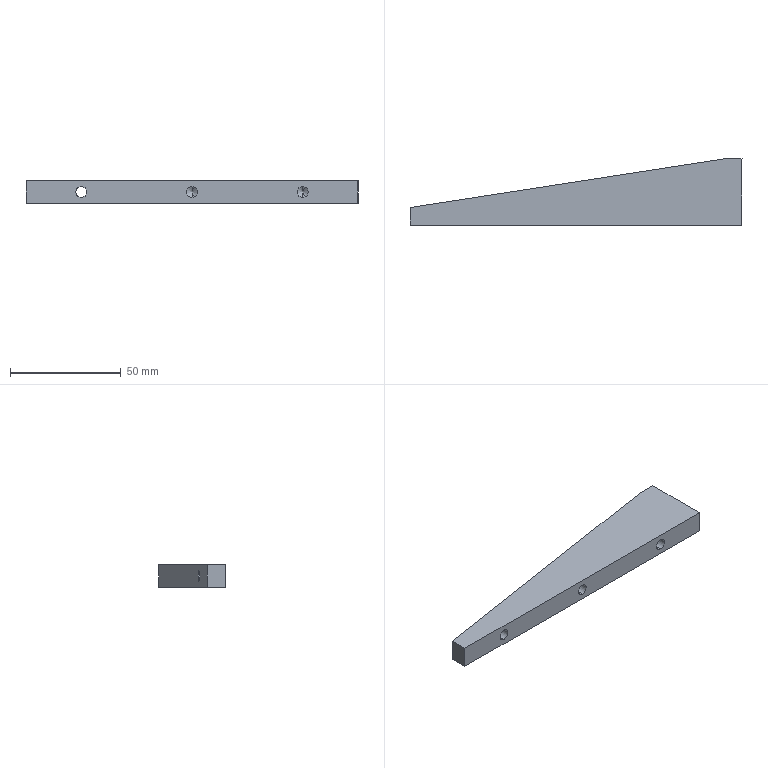Component | SolidWorks | 17081801-804-026A-1 | 1 solid | 25 faces | box 150 x 30 x 10 mm | volume 27929 mm3 | cylinder 10 | cone 8 | plane 7 | commonest cylinder face diameters 5 x10 | material AL6061
build123d program:
from build123d import *

# Parameters (mm, degrees)
BOSS_EXTRUDE1_DEPTH   = 5
M6_TAPPED_HOLE1_D     = 5
M6_TAPPED_HOLE1_DEPTH = 15
M6_TAPPED_HOLE1_TIP   = 1.502
M6_TAPPED_HOLE2_D     = 5
M6_TAPPED_HOLE2_DEPTH = 15
M6_TAPPED_HOLE2_TIP   = 1.502


with BuildPart() as part:
    # Sketch1 → Boss-Extrude1 (new, symmetric)
    with BuildSketch(Plane.XY):
        Polygon((0, 0), (0, 150), (-8, 150), (-30, 8), (-30, 0), align=None)
    extrude(amount=BOSS_EXTRUDE1_DEPTH, both=True)

    # M6 Tapped Hole1
    with Locations(Plane(origin=(0, 0, 0), x_dir=(0, 0, -1), z_dir=(1, 0, 0))):
        with Locations((0, 25), (0, 75), (0, 125)):
            Hole(M6_TAPPED_HOLE1_D / 2, depth=M6_TAPPED_HOLE1_DEPTH)
            with Locations((0, 0, -(M6_TAPPED_HOLE1_DEPTH + M6_TAPPED_HOLE1_TIP / 2))):  # 118° drill point
                Cone(0, M6_TAPPED_HOLE1_D / 2, M6_TAPPED_HOLE1_TIP, mode=Mode.SUBTRACT)

    # M6 Tapped Hole2
    with Locations(Plane(origin=(0, 0, 0), x_dir=(-1, 0, 0), z_dir=(0, -1, 0))):
        with Locations((25, 0), (10, 0)):
            Hole(M6_TAPPED_HOLE2_D / 2, depth=M6_TAPPED_HOLE2_DEPTH)
            with Locations((0, 0, -(M6_TAPPED_HOLE2_DEPTH + M6_TAPPED_HOLE2_TIP / 2))):  # 118° drill point
                Cone(0, M6_TAPPED_HOLE2_D / 2, M6_TAPPED_HOLE2_TIP, mode=Mode.SUBTRACT)


solid = part.part

# Placed as in the assembly
solid = solid.moved(Location((237, 2110.4, 171), (180, 0, 90)))
STEP:
#1=CARTESIAN_POINT('',(8.74,84.071,6.634));
#2=VERTEX_POINT('',#1);
#3=CARTESIAN_POINT('',(8.74,84.071,6.831));
#4=VERTEX_POINT('',#3);
#5=CARTESIAN_POINT('',(8.74,84.071,6.732));
#6=DIRECTION('',(1.,-0.,0.));
#7=DIRECTION('',(0.,0.,1.));
#8=AXIS2_PLACEMENT_3D('',#5,#6,#7);
#9=CIRCLE('',#8,0.09843);
#10=EDGE_CURVE('',#2,#4,#9,.T.);
#11=ORIENTED_EDGE('',*,*,#10,.F.);
#12=CARTESIAN_POINT('',(9.331,84.071,6.634));
#13=VERTEX_POINT('',#12);
#14=CARTESIAN_POINT('',(9.331,84.071,6.634));
#15=DIRECTION('',(1.,-0.,0.));
#16=VECTOR('',#15,39.37);
#17=LINE('',#14,#16);
#18=EDGE_CURVE('',#2,#13,#17,.T.);
#19=ORIENTED_EDGE('',*,*,#18,.T.);
#20=CARTESIAN_POINT('',(9.331,84.071,6.831));
#21=VERTEX_POINT('',#20);
#22=CARTESIAN_POINT('',(9.331,84.071,6.732));
#23=DIRECTION('',(1.,-0.,0.));
#24=DIRECTION('',(0.,0.,1.));
#25=AXIS2_PLACEMENT_3D('',#22,#23,#24);
#26=CIRCLE('',#25,0.09843);
#27=EDGE_CURVE('',#13,#21,#26,.T.);
#28=ORIENTED_EDGE('',*,*,#27,.T.);
#29=CARTESIAN_POINT('',(9.331,84.071,6.831));
#30=DIRECTION('',(1.,-0.,0.));
#31=VECTOR('',#30,39.37);
#32=LINE('',#29,#31);
#33=EDGE_CURVE('',#4,#21,#32,.T.);
#34=ORIENTED_EDGE('',*,*,#33,.F.);
#35=EDGE_LOOP('',(#11,#19,#28,#34));
#36=FACE_OUTER_BOUND('',#35,.T.);
#37=CARTESIAN_POINT('',(9.331,84.071,6.732));
#38=DIRECTION('',(1.,-0.,0.));
#39=DIRECTION('',(0.,0.,1.));
#40=AXIS2_PLACEMENT_3D('',#37,#38,#39);
#41=CYLINDRICAL_SURFACE('',#40,0.09843);
#42=ADVANCED_FACE('',(#36),#41,.F.);
#43=CARTESIAN_POINT('',(8.681,84.071,6.732));
#44=VERTEX_POINT('',#43);
#45=CARTESIAN_POINT('',(8.74,84.071,6.831));
#46=DIRECTION('',(0.515,-0.,0.8572));
#47=VECTOR('',#46,39.37);
#48=LINE('',#45,#47);
#49=EDGE_CURVE('',#44,#4,#48,.T.);
#50=ORIENTED_EDGE('',*,*,#49,.F.);
#51=CARTESIAN_POINT('',(8.74,84.071,6.634));
#52=DIRECTION('',(0.515,-0.,-0.8572));
#53=VECTOR('',#52,39.37);
#54=LINE('',#51,#53);
#55=EDGE_CURVE('',#44,#2,#54,.T.);
#56=ORIENTED_EDGE('',*,*,#55,.T.);
#57=ORIENTED_EDGE('',*,*,#10,.T.);
#58=EDGE_LOOP('',(#50,#56,#57));
#59=FACE_OUTER_BOUND('',#58,.T.);
#60=CARTESIAN_POINT('',(8.74,84.071,6.732));
#61=DIRECTION('',(1.,-0.,0.));
#62=DIRECTION('',(0.,0.,1.));
#63=AXIS2_PLACEMENT_3D('',#60,#61,#62);
#64=CONICAL_SURFACE('',#63,0.09843,1.03);
#65=ADVANCED_FACE('',(#59),#64,.F.);
#66=CARTESIAN_POINT('',(8.74,83.48,6.634));
#67=VERTEX_POINT('',#66);
#68=CARTESIAN_POINT('',(8.74,83.48,6.831));
#69=VERTEX_POINT('',#68);
#70=CARTESIAN_POINT('',(8.74,83.48,6.732));
#71=DIRECTION('',(1.,-0.,0.));
#72=DIRECTION('',(0.,0.,1.));
#73=AXIS2_PLACEMENT_3D('',#70,#71,#72);
#74=CIRCLE('',#73,0.09843);
#75=EDGE_CURVE('',#67,#69,#74,.T.);
#76=ORIENTED_EDGE('',*,*,#75,.F.);
#77=CARTESIAN_POINT('',(9.331,83.48,6.634));
#78=VERTEX_POINT('',#77);
#79=CARTESIAN_POINT('',(9.331,83.48,6.634));
#80=DIRECTION('',(1.,-0.,0.));
#81=VECTOR('',#80,39.37);
#82=LINE('',#79,#81);
#83=EDGE_CURVE('',#67,#78,#82,.T.);
#84=ORIENTED_EDGE('',*,*,#83,.T.);
#85=CARTESIAN_POINT('',(9.331,83.48,6.831));
#86=VERTEX_POINT('',#85);
#87=CARTESIAN_POINT('',(9.331,83.48,6.732));
#88=DIRECTION('',(1.,-0.,0.));
#89=DIRECTION('',(0.,0.,1.));
#90=AXIS2_PLACEMENT_3D('',#87,#88,#89);
#91=CIRCLE('',#90,0.09843);
#92=EDGE_CURVE('',#78,#86,#91,.T.);
#93=ORIENTED_EDGE('',*,*,#92,.T.);
#94=CARTESIAN_POINT('',(9.331,83.48,6.831));
#95=DIRECTION('',(1.,-0.,0.));
#96=VECTOR('',#95,39.37);
#97=LINE('',#94,#96);
#98=EDGE_CURVE('',#69,#86,#97,.T.);
#99=ORIENTED_EDGE('',*,*,#98,.F.);
#100=EDGE_LOOP('',(#76,#84,#93,#99));
#101=FACE_OUTER_BOUND('',#100,.T.);
#102=CARTESIAN_POINT('',(9.331,83.48,6.732));
#103=DIRECTION('',(1.,-0.,0.));
#104=DIRECTION('',(0.,0.,1.));
#105=AXIS2_PLACEMENT_3D('',#102,#103,#104);
#106=CYLINDRICAL_SURFACE('',#105,0.09843);
#107=ADVANCED_FACE('',(#101),#106,.F.);
#108=CARTESIAN_POINT('',(8.681,83.48,6.732));
#109=VERTEX_POINT('',#108);
#110=CARTESIAN_POINT('',(8.74,83.48,6.831));
#111=DIRECTION('',(0.515,-0.,0.8572));
#112=VECTOR('',#111,39.37);
#113=LINE('',#110,#112);
#114=EDGE_CURVE('',#109,#69,#113,.T.);
#115=ORIENTED_EDGE('',*,*,#114,.F.);
#116=CARTESIAN_POINT('',(8.74,83.48,6.634));
#117=DIRECTION('',(0.515,-0.,-0.8572));
#118=VECTOR('',#117,39.37);
#119=LINE('',#116,#118);
#120=EDGE_CURVE('',#109,#67,#119,.T.);
#121=ORIENTED_EDGE('',*,*,#120,.T.);
#122=ORIENTED_EDGE('',*,*,#75,.T.);
#123=EDGE_LOOP('',(#115,#121,#122));
#124=FACE_OUTER_BOUND('',#123,.T.);
#125=CARTESIAN_POINT('',(8.74,83.48,6.732));
#126=DIRECTION('',(1.,-0.,0.));
#127=DIRECTION('',(0.,0.,1.));
#128=AXIS2_PLACEMENT_3D('',#125,#126,#127);
#129=CONICAL_SURFACE('',#128,0.09843,1.03);
#130=ADVANCED_FACE('',(#124),#129,.F.);
#131=CARTESIAN_POINT('',(8.346,83.677,6.634));
#132=VERTEX_POINT('',#131);
#133=CARTESIAN_POINT('',(8.346,83.677,6.831));
#134=VERTEX_POINT('',#133);
#135=CARTESIAN_POINT('',(8.346,83.677,6.732));
#136=DIRECTION('',(-0.,-1.,-0.));
#137=DIRECTION('',(0.,0.,1.));
#138=AXIS2_PLACEMENT_3D('',#135,#136,#137);
#139=CIRCLE('',#138,0.09843);
#140=EDGE_CURVE('',#132,#134,#139,.T.);
#141=ORIENTED_EDGE('',*,*,#140,.F.);
#142=CARTESIAN_POINT('',(8.346,83.087,6.634));
#143=VERTEX_POINT('',#142);
#144=CARTESIAN_POINT('',(8.346,83.087,6.634));
#145=DIRECTION('',(-0.,-1.,-0.));
#146=VECTOR('',#145,39.37);
#147=LINE('',#144,#146);
#148=EDGE_CURVE('',#132,#143,#147,.T.);
#149=ORIENTED_EDGE('',*,*,#148,.T.);
#150=CARTESIAN_POINT('',(8.346,83.087,6.831));
#151=VERTEX_POINT('',#150);
#152=CARTESIAN_POINT('',(8.346,83.087,6.732));
#153=DIRECTION('',(-0.,-1.,-0.));
#154=DIRECTION('',(0.,0.,1.));
#155=AXIS2_PLACEMENT_3D('',#152,#153,#154);
#156=CIRCLE('',#155,0.09843);
#157=EDGE_CURVE('',#143,#151,#156,.T.);
#158=ORIENTED_EDGE('',*,*,#157,.T.);
#159=CARTESIAN_POINT('',(8.346,83.087,6.831));
#160=DIRECTION('',(-0.,-1.,-0.));
#161=VECTOR('',#160,39.37);
#162=LINE('',#159,#161);
#163=EDGE_CURVE('',#134,#151,#162,.T.);
#164=ORIENTED_EDGE('',*,*,#163,.F.);
#165=EDGE_LOOP('',(#141,#149,#158,#164));
#166=FACE_OUTER_BOUND('',#165,.T.);
#167=CARTESIAN_POINT('',(8.346,83.087,6.732));
#168=DIRECTION('',(-0.,-1.,-0.));
#169=DIRECTION('',(0.,0.,1.));
#170=AXIS2_PLACEMENT_3D('',#167,#168,#169);
#171=CYLINDRICAL_SURFACE('',#170,0.09843);
#172=ADVANCED_FACE('',(#166),#171,.F.);
#173=CARTESIAN_POINT('',(8.346,83.736,6.732));
#174=VERTEX_POINT('',#173);
#175=CARTESIAN_POINT('',(8.346,83.677,6.831));
#176=DIRECTION('',(-0.,-0.515,0.8572));
#177=VECTOR('',#176,39.37);
#178=LINE('',#175,#177);
#179=EDGE_CURVE('',#174,#134,#178,.T.);
#180=ORIENTED_EDGE('',*,*,#179,.F.);
#181=CARTESIAN_POINT('',(8.346,83.677,6.634));
#182=DIRECTION('',(-0.,-0.515,-0.8572));
#183=VECTOR('',#182,39.37);
#184=LINE('',#181,#183);
#185=EDGE_CURVE('',#174,#132,#184,.T.);
#186=ORIENTED_EDGE('',*,*,#185,.T.);
#187=ORIENTED_EDGE('',*,*,#140,.T.);
#188=EDGE_LOOP('',(#180,#186,#187));
#189=FACE_OUTER_BOUND('',#188,.T.);
#190=CARTESIAN_POINT('',(8.346,83.677,6.732));
#191=DIRECTION('',(-0.,-1.,-0.));
#192=DIRECTION('',(0.,0.,1.));
#193=AXIS2_PLACEMENT_3D('',#190,#191,#192);
#194=CONICAL_SURFACE('',#193,0.09843,1.03);
#195=ADVANCED_FACE('',(#189),#194,.F.);
#196=CARTESIAN_POINT('',(6.378,83.677,6.634));
#197=VERTEX_POINT('',#196);
#198=CARTESIAN_POINT('',(6.378,83.677,6.831));
#199=VERTEX_POINT('',#198);
#200=CARTESIAN_POINT('',(6.378,83.677,6.732));
#201=DIRECTION('',(-0.,-1.,-0.));
#202=DIRECTION('',(0.,0.,1.));
#203=AXIS2_PLACEMENT_3D('',#200,#201,#202);
#204=CIRCLE('',#203,0.09843);
#205=EDGE_CURVE('',#197,#199,#204,.T.);
#206=ORIENTED_EDGE('',*,*,#205,.F.);
#207=CARTESIAN_POINT('',(6.378,83.087,6.634));
#208=VERTEX_POINT('',#207);
#209=CARTESIAN_POINT('',(6.378,83.087,6.634));
#210=DIRECTION('',(-0.,-1.,-0.));
#211=VECTOR('',#210,39.37);
#212=LINE('',#209,#211);
#213=EDGE_CURVE('',#197,#208,#212,.T.);
#214=ORIENTED_EDGE('',*,*,#213,.T.);
#215=CARTESIAN_POINT('',(6.378,83.087,6.831));
#216=VERTEX_POINT('',#215);
#217=CARTESIAN_POINT('',(6.378,83.087,6.732));
#218=DIRECTION('',(-0.,-1.,-0.));
#219=DIRECTION('',(0.,0.,1.));
#220=AXIS2_PLACEMENT_3D('',#217,#218,#219);
#221=CIRCLE('',#220,0.09843);
#222=EDGE_CURVE('',#208,#216,#221,.T.);
#223=ORIENTED_EDGE('',*,*,#222,.T.);
#224=CARTESIAN_POINT('',(6.378,83.087,6.831));
#225=DIRECTION('',(-0.,-1.,-0.));
#226=VECTOR('',#225,39.37);
#227=LINE('',#224,#226);
#228=EDGE_CURVE('',#199,#216,#227,.T.);
#229=ORIENTED_EDGE('',*,*,#228,.F.);
#230=EDGE_LOOP('',(#206,#214,#223,#229));
#231=FACE_OUTER_BOUND('',#230,.T.);
#232=CARTESIAN_POINT('',(6.378,83.087,6.732));
#233=DIRECTION('',(-0.,-1.,-0.));
#234=DIRECTION('',(0.,0.,1.));
#235=AXIS2_PLACEMENT_3D('',#232,#233,#234);
#236=CYLINDRICAL_SURFACE('',#235,0.09843);
#237=ADVANCED_FACE('',(#231),#236,.F.);
#238=CARTESIAN_POINT('',(6.378,83.736,6.732));
#239=VERTEX_POINT('',#238);
#240=CARTESIAN_POINT('',(6.378,83.677,6.831));
#241=DIRECTION('',(-0.,-0.515,0.8572));
#242=VECTOR('',#241,39.37);
#243=LINE('',#240,#242);
#244=EDGE_CURVE('',#239,#199,#243,.T.);
#245=ORIENTED_EDGE('',*,*,#244,.F.);
#246=CARTESIAN_POINT('',(6.378,83.677,6.634));
#247=DIRECTION('',(-0.,-0.515,-0.8572));
#248=VECTOR('',#247,39.37);
#249=LINE('',#246,#248);
#250=EDGE_CURVE('',#239,#197,#249,.T.);
#251=ORIENTED_EDGE('',*,*,#250,.T.);
#252=ORIENTED_EDGE('',*,*,#205,.T.);
#253=EDGE_LOOP('',(#245,#251,#252));
#254=FACE_OUTER_BOUND('',#253,.T.);
#255=CARTESIAN_POINT('',(6.378,83.677,6.732));
#256=DIRECTION('',(-0.,-1.,-0.));
#257=DIRECTION('',(0.,0.,1.));
#258=AXIS2_PLACEMENT_3D('',#255,#256,#257);
#259=CONICAL_SURFACE('',#258,0.09843,1.03);
#260=ADVANCED_FACE('',(#254),#259,.F.);
#261=CARTESIAN_POINT('',(4.409,83.554,6.634));
#262=VERTEX_POINT('',#261);
#263=CARTESIAN_POINT('',(4.409,83.554,6.831));
#264=VERTEX_POINT('',#263);
#265=CARTESIAN_POINT('',(4.409,83.554,6.634));
#266=CARTESIAN_POINT('',(4.606,83.585,6.634));
#267=CARTESIAN_POINT('',(4.606,83.585,6.831));
#268=CARTESIAN_POINT('',(4.409,83.554,6.831));
#269=(BOUNDED_CURVE()B_SPLINE_CURVE(3,(#265,#266,#267,#268),.UNSPECIFIED.,.F.,.T.)B_SPLINE_CURVE_WITH_KNOTS((4,4),(1.571,4.712),.UNSPECIFIED.)CURVE()GEOMETRIC_REPRESENTATION_ITEM()RATIONAL_B_SPLINE_CURVE((1.,0.3333,0.3333,1.))REPRESENTATION_ITEM(''));
#270=EDGE_CURVE('',#262,#264,#269,.T.);
#271=ORIENTED_EDGE('',*,*,#270,.F.);
#272=CARTESIAN_POINT('',(4.409,83.087,6.634));
#273=VERTEX_POINT('',#272);
#274=CARTESIAN_POINT('',(4.409,83.087,6.634));
#275=DIRECTION('',(-0.,-1.,-0.));
#276=VECTOR('',#275,39.37);
#277=LINE('',#274,#276);
#278=EDGE_CURVE('',#262,#273,#277,.T.);
#279=ORIENTED_EDGE('',*,*,#278,.T.);
#280=CARTESIAN_POINT('',(4.409,83.087,6.831));
#281=VERTEX_POINT('',#280);
#282=CARTESIAN_POINT('',(4.409,83.087,6.732));
#283=DIRECTION('',(-0.,-1.,-0.));
#284=DIRECTION('',(0.,0.,1.));
#285=AXIS2_PLACEMENT_3D('',#282,#283,#284);
#286=CIRCLE('',#285,0.09843);
#287=EDGE_CURVE('',#273,#281,#286,.T.);
#288=ORIENTED_EDGE('',*,*,#287,.T.);
#289=CARTESIAN_POINT('',(4.409,83.087,6.831));
#290=DIRECTION('',(-0.,-1.,-0.));
#291=VECTOR('',#290,39.37);
#292=LINE('',#289,#291);
#293=EDGE_CURVE('',#264,#281,#292,.T.);
#294=ORIENTED_EDGE('',*,*,#293,.F.);
#295=EDGE_LOOP('',(#271,#279,#288,#294));
#296=FACE_OUTER_BOUND('',#295,.T.);
#297=CARTESIAN_POINT('',(4.409,83.087,6.732));
#298=DIRECTION('',(-0.,-1.,-0.));
#299=DIRECTION('',(0.,0.,1.));
#300=AXIS2_PLACEMENT_3D('',#297,#298,#299);
#301=CYLINDRICAL_SURFACE('',#300,0.09843);
#302=ADVANCED_FACE('',(#296),#301,.F.);
#303=CARTESIAN_POINT('',(9.331,84.071,6.732));
#304=DIRECTION('',(1.,-0.,0.));
#305=DIRECTION('',(0.,0.,1.));
#306=AXIS2_PLACEMENT_3D('',#303,#304,#305);
#307=CIRCLE('',#306,0.09843);
#308=EDGE_CURVE('',#21,#13,#307,.T.);
#309=ORIENTED_EDGE('',*,*,#308,.F.);
#310=ORIENTED_EDGE('',*,*,#27,.F.);
#311=EDGE_LOOP('',(#309,#310));
#312=FACE_BOUND('',#311,.T.);
#313=CARTESIAN_POINT('',(9.331,83.48,6.732));
#314=DIRECTION('',(1.,-0.,0.));
#315=DIRECTION('',(0.,0.,1.));
#316=AXIS2_PLACEMENT_3D('',#313,#314,#315);
#317=CIRCLE('',#316,0.09843);
#318=EDGE_CURVE('',#86,#78,#317,.T.);
#319=ORIENTED_EDGE('',*,*,#318,.F.);
#320=ORIENTED_EDGE('',*,*,#92,.F.);
#321=EDGE_LOOP('',(#319,#320));
#322=FACE_BOUND('',#321,.T.);
#323=CARTESIAN_POINT('',(9.331,84.268,6.929));
#324=VERTEX_POINT('',#323);
#325=CARTESIAN_POINT('',(9.331,83.087,6.929));
#326=VERTEX_POINT('',#325);
#327=CARTESIAN_POINT('',(9.331,84.268,6.929));
#328=DIRECTION('',(-0.,-1.,-0.));
#329=VECTOR('',#328,39.37);
#330=LINE('',#327,#329);
#331=EDGE_CURVE('',#324,#326,#330,.T.);
#332=ORIENTED_EDGE('',*,*,#331,.T.);
#333=CARTESIAN_POINT('',(9.331,83.087,6.535));
#334=VERTEX_POINT('',#333);
#335=CARTESIAN_POINT('',(9.331,83.087,6.535));
#336=DIRECTION('',(-0.,-0.,1.));
#337=VECTOR('',#336,39.37);
#338=LINE('',#335,#337);
#339=EDGE_CURVE('',#334,#326,#338,.T.);
#340=ORIENTED_EDGE('',*,*,#339,.F.);
#341=CARTESIAN_POINT('',(9.331,84.268,6.535));
#342=VERTEX_POINT('',#341);
#343=CARTESIAN_POINT('',(9.331,84.268,6.535));
#344=DIRECTION('',(-0.,-1.,-0.));
#345=VECTOR('',#344,39.37);
#346=LINE('',#343,#345);
#347=EDGE_CURVE('',#342,#334,#346,.T.);
#348=ORIENTED_EDGE('',*,*,#347,.F.);
#349=CARTESIAN_POINT('',(9.331,84.268,6.535));
#350=DIRECTION('',(-0.,-0.,1.));
#351=VECTOR('',#350,39.37);
#352=LINE('',#349,#351);
#353=EDGE_CURVE('',#342,#324,#352,.T.);
#354=ORIENTED_EDGE('',*,*,#353,.T.);
#355=EDGE_LOOP('',(#332,#340,#348,#354));
#356=FACE_OUTER_BOUND('',#355,.T.);
#357=CARTESIAN_POINT('',(9.331,84.268,6.535));
#358=DIRECTION('',(-1.,0.,-0.));
#359=DIRECTION('',(0.,0.,-1.));
#360=AXIS2_PLACEMENT_3D('',#357,#358,#359);
#361=PLANE('',#360);
#362=ADVANCED_FACE('',(#312,#322,#356),#361,.F.);
#363=CARTESIAN_POINT('',(8.346,83.087,6.732));
#364=DIRECTION('',(-0.,-1.,-0.));
#365=DIRECTION('',(0.,0.,1.));
#366=AXIS2_PLACEMENT_3D('',#363,#364,#365);
#367=CIRCLE('',#366,0.09843);
#368=EDGE_CURVE('',#151,#143,#367,.T.);
#369=ORIENTED_EDGE('',*,*,#368,.F.);
#370=ORIENTED_EDGE('',*,*,#157,.F.);
#371=EDGE_LOOP('',(#369,#370));
#372=FACE_BOUND('',#371,.T.);
#373=CARTESIAN_POINT('',(6.378,83.087,6.732));
#374=DIRECTION('',(-0.,-1.,-0.));
#375=DIRECTION('',(0.,0.,1.));
#376=AXIS2_PLACEMENT_3D('',#373,#374,#375);
#377=CIRCLE('',#376,0.09843);
#378=EDGE_CURVE('',#216,#208,#377,.T.);
#379=ORIENTED_EDGE('',*,*,#378,.F.);
#380=ORIENTED_EDGE('',*,*,#222,.F.);
#381=EDGE_LOOP('',(#379,#380));
#382=FACE_BOUND('',#381,.T.);
#383=CARTESIAN_POINT('',(4.409,83.087,6.732));
#384=DIRECTION('',(-0.,-1.,-0.));
#385=DIRECTION('',(0.,0.,1.));
#386=AXIS2_PLACEMENT_3D('',#383,#384,#385);
#387=CIRCLE('',#386,0.09843);
#388=EDGE_CURVE('',#281,#273,#387,.T.);
#389=ORIENTED_EDGE('',*,*,#388,.F.);
#390=ORIENTED_EDGE('',*,*,#287,.F.);
#391=EDGE_LOOP('',(#389,#390));
#392=FACE_BOUND('',#391,.T.);
#393=CARTESIAN_POINT('',(3.425,83.087,6.929));
#394=VERTEX_POINT('',#393);
#395=CARTESIAN_POINT('',(9.331,83.087,6.929));
#396=DIRECTION('',(-1.,0.,-0.));
#397=VECTOR('',#396,39.37);
#398=LINE('',#395,#397);
#399=EDGE_CURVE('',#326,#394,#398,.T.);
#400=ORIENTED_EDGE('',*,*,#399,.T.);
#401=CARTESIAN_POINT('',(3.425,83.087,6.535));
#402=VERTEX_POINT('',#401);
#403=CARTESIAN_POINT('',(3.425,83.087,6.535));
#404=DIRECTION('',(-0.,-0.,1.));
#405=VECTOR('',#404,39.37);
#406=LINE('',#403,#405);
#407=EDGE_CURVE('',#402,#394,#406,.T.);
#408=ORIENTED_EDGE('',*,*,#407,.F.);
#409=CARTESIAN_POINT('',(9.331,83.087,6.535));
#410=DIRECTION('',(-1.,0.,-0.));
#411=VECTOR('',#410,39.37);
#412=LINE('',#409,#411);
#413=EDGE_CURVE('',#334,#402,#412,.T.);
#414=ORIENTED_EDGE('',*,*,#413,.F.);
#415=ORIENTED_EDGE('',*,*,#339,.T.);
#416=EDGE_LOOP('',(#400,#408,#414,#415));
#417=FACE_OUTER_BOUND('',#416,.T.);
#418=CARTESIAN_POINT('',(9.331,83.087,6.535));
#419=DIRECTION('',(0.,1.,0.));
#420=DIRECTION('',(0.,0.,-1.));
#421=AXIS2_PLACEMENT_3D('',#418,#419,#420);
#422=PLANE('',#421);
#423=ADVANCED_FACE('',(#372,#382,#392,#417),#422,.F.);
#424=CARTESIAN_POINT('',(3.425,83.402,6.929));
#425=VERTEX_POINT('',#424);
#426=CARTESIAN_POINT('',(3.425,83.087,6.929));
#427=DIRECTION('',(0.,1.,0.));
#428=VECTOR('',#427,39.37);
#429=LINE('',#426,#428);
#430=EDGE_CURVE('',#394,#425,#429,.T.);
#431=ORIENTED_EDGE('',*,*,#430,.T.);
#432=CARTESIAN_POINT('',(3.425,83.402,6.535));
#433=VERTEX_POINT('',#432);
#434=CARTESIAN_POINT('',(3.425,83.402,6.535));
#435=DIRECTION('',(-0.,-0.,1.));
#436=VECTOR('',#435,39.37);
#437=LINE('',#434,#436);
#438=EDGE_CURVE('',#433,#425,#437,.T.);
#439=ORIENTED_EDGE('',*,*,#438,.F.);
#440=CARTESIAN_POINT('',(3.425,83.087,6.535));
#441=DIRECTION('',(0.,1.,0.));
#442=VECTOR('',#441,39.37);
#443=LINE('',#440,#442);
#444=EDGE_CURVE('',#402,#433,#443,.T.);
#445=ORIENTED_EDGE('',*,*,#444,.F.);
#446=ORIENTED_EDGE('',*,*,#407,.T.);
#447=EDGE_LOOP('',(#431,#439,#445,#446));
#448=FACE_OUTER_BOUND('',#447,.T.);
#449=CARTESIAN_POINT('',(3.425,83.087,6.535));
#450=DIRECTION('',(1.,-0.,0.));
#451=DIRECTION('',(-0.,-0.,1.));
#452=AXIS2_PLACEMENT_3D('',#449,#450,#451);
#453=PLANE('',#452);
#454=ADVANCED_FACE('',(#448),#453,.F.);
#455=CARTESIAN_POINT('',(4.409,83.554,6.831));
#456=CARTESIAN_POINT('',(4.213,83.524,6.831));
#457=CARTESIAN_POINT('',(4.213,83.524,6.634));
#458=CARTESIAN_POINT('',(4.409,83.554,6.634));
#459=(BOUNDED_CURVE()B_SPLINE_CURVE(3,(#455,#456,#457,#458),.UNSPECIFIED.,.F.,.F.)B_SPLINE_CURVE_WITH_KNOTS((4,4),(4.712,7.854),.UNSPECIFIED.)CURVE()GEOMETRIC_REPRESENTATION_ITEM()RATIONAL_B_SPLINE_CURVE((1.,0.3333,0.3333,1.))REPRESENTATION_ITEM(''));
#460=EDGE_CURVE('',#264,#262,#459,.T.);
#461=ORIENTED_EDGE('',*,*,#460,.T.);
#462=ORIENTED_EDGE('',*,*,#270,.T.);
#463=EDGE_LOOP('',(#461,#462));
#464=FACE_BOUND('',#463,.T.);
#465=CARTESIAN_POINT('',(9.016,84.268,6.929));
#466=VERTEX_POINT('',#465);
#467=CARTESIAN_POINT('',(3.425,83.402,6.929));
#468=DIRECTION('',(0.9882,0.1531,0.));
#469=VECTOR('',#468,39.37);
#470=LINE('',#467,#469);
#471=EDGE_CURVE('',#425,#466,#470,.T.);
#472=ORIENTED_EDGE('',*,*,#471,.T.);
#473=CARTESIAN_POINT('',(9.016,84.268,6.535));
#474=VERTEX_POINT('',#473);
#475=CARTESIAN_POINT('',(9.016,84.268,6.535));
#476=DIRECTION('',(-0.,-0.,1.));
#477=VECTOR('',#476,39.37);
#478=LINE('',#475,#477);
#479=EDGE_CURVE('',#474,#466,#478,.T.);
#480=ORIENTED_EDGE('',*,*,#479,.F.);
#481=CARTESIAN_POINT('',(3.425,83.402,6.535));
#482=DIRECTION('',(0.9882,0.1531,0.));
#483=VECTOR('',#482,39.37);
#484=LINE('',#481,#483);
#485=EDGE_CURVE('',#433,#474,#484,.T.);
#486=ORIENTED_EDGE('',*,*,#485,.F.);
#487=ORIENTED_EDGE('',*,*,#438,.T.);
#488=EDGE_LOOP('',(#472,#480,#486,#487));
#489=FACE_OUTER_BOUND('',#488,.T.);
#490=CARTESIAN_POINT('',(3.425,83.402,6.535));
#491=DIRECTION('',(0.1531,-0.9882,-0.));
#492=DIRECTION('',(-0.9882,-0.1531,-0.));
#493=AXIS2_PLACEMENT_3D('',#490,#491,#492);
#494=PLANE('',#493);
#495=ADVANCED_FACE('',(#464,#489),#494,.F.);
#496=CARTESIAN_POINT('',(9.016,84.268,6.929));
#497=DIRECTION('',(1.,-0.,0.));
#498=VECTOR('',#497,39.37);
#499=LINE('',#496,#498);
#500=EDGE_CURVE('',#466,#324,#499,.T.);
#501=ORIENTED_EDGE('',*,*,#500,.T.);
#502=ORIENTED_EDGE('',*,*,#353,.F.);
#503=CARTESIAN_POINT('',(9.016,84.268,6.535));
#504=DIRECTION('',(1.,-0.,0.));
#505=VECTOR('',#504,39.37);
#506=LINE('',#503,#505);
#507=EDGE_CURVE('',#474,#342,#506,.T.);
#508=ORIENTED_EDGE('',*,*,#507,.F.);
#509=ORIENTED_EDGE('',*,*,#479,.T.);
#510=EDGE_LOOP('',(#501,#502,#508,#509));
#511=FACE_OUTER_BOUND('',#510,.T.);
#512=CARTESIAN_POINT('',(9.016,84.268,6.535));
#513=DIRECTION('',(-0.,-1.,-0.));
#514=DIRECTION('',(-0.,-0.,1.));
#515=AXIS2_PLACEMENT_3D('',#512,#513,#514);
#516=PLANE('',#515);
#517=ADVANCED_FACE('',(#511),#516,.F.);
#518=ORIENTED_EDGE('',*,*,#347,.T.);
#519=ORIENTED_EDGE('',*,*,#413,.T.);
#520=ORIENTED_EDGE('',*,*,#444,.T.);
#521=ORIENTED_EDGE('',*,*,#485,.T.);
#522=ORIENTED_EDGE('',*,*,#507,.T.);
#523=EDGE_LOOP('',(#518,#519,#520,#521,#522));
#524=FACE_OUTER_BOUND('',#523,.T.);
#525=CARTESIAN_POINT('',(9.331,83.087,6.535));
#526=DIRECTION('',(0.,0.,-1.));
#527=DIRECTION('',(-0.,-1.,-0.));
#528=AXIS2_PLACEMENT_3D('',#525,#526,#527);
#529=PLANE('',#528);
#530=ADVANCED_FACE('',(#524),#529,.T.);
#531=ORIENTED_EDGE('',*,*,#331,.F.);
#532=ORIENTED_EDGE('',*,*,#500,.F.);
#533=ORIENTED_EDGE('',*,*,#471,.F.);
#534=ORIENTED_EDGE('',*,*,#430,.F.);
#535=ORIENTED_EDGE('',*,*,#399,.F.);
#536=EDGE_LOOP('',(#531,#532,#533,#534,#535));
#537=FACE_OUTER_BOUND('',#536,.T.);
#538=CARTESIAN_POINT('',(9.331,83.087,6.929));
#539=DIRECTION('',(0.,0.,-1.));
#540=DIRECTION('',(-0.,-1.,-0.));
#541=AXIS2_PLACEMENT_3D('',#538,#539,#540);
#542=PLANE('',#541);
#543=ADVANCED_FACE('',(#537),#542,.F.);
#544=ORIENTED_EDGE('',*,*,#278,.F.);
#545=ORIENTED_EDGE('',*,*,#460,.F.);
#546=ORIENTED_EDGE('',*,*,#293,.T.);
#547=ORIENTED_EDGE('',*,*,#388,.T.);
#548=EDGE_LOOP('',(#544,#545,#546,#547));
#549=FACE_OUTER_BOUND('',#548,.T.);
#550=CARTESIAN_POINT('',(4.409,83.087,6.732));
#551=DIRECTION('',(-0.,-1.,-0.));
#552=DIRECTION('',(0.,0.,1.));
#553=AXIS2_PLACEMENT_3D('',#550,#551,#552);
#554=CYLINDRICAL_SURFACE('',#553,0.09843);
#555=ADVANCED_FACE('',(#549),#554,.F.);
#556=ORIENTED_EDGE('',*,*,#250,.F.);
#557=ORIENTED_EDGE('',*,*,#244,.T.);
#558=CARTESIAN_POINT('',(6.378,83.677,6.732));
#559=DIRECTION('',(-0.,-1.,-0.));
#560=DIRECTION('',(0.,0.,1.));
#561=AXIS2_PLACEMENT_3D('',#558,#559,#560);
#562=CIRCLE('',#561,0.09843);
#563=EDGE_CURVE('',#199,#197,#562,.T.);
#564=ORIENTED_EDGE('',*,*,#563,.T.);
#565=EDGE_LOOP('',(#556,#557,#564));
#566=FACE_OUTER_BOUND('',#565,.T.);
#567=CARTESIAN_POINT('',(6.378,83.677,6.732));
#568=DIRECTION('',(-0.,-1.,-0.));
#569=DIRECTION('',(0.,0.,1.));
#570=AXIS2_PLACEMENT_3D('',#567,#568,#569);
#571=CONICAL_SURFACE('',#570,0.09843,1.03);
#572=ADVANCED_FACE('',(#566),#571,.F.);
#573=ORIENTED_EDGE('',*,*,#213,.F.);
#574=ORIENTED_EDGE('',*,*,#563,.F.);
#575=ORIENTED_EDGE('',*,*,#228,.T.);
#576=ORIENTED_EDGE('',*,*,#378,.T.);
#577=EDGE_LOOP('',(#573,#574,#575,#576));
#578=FACE_OUTER_BOUND('',#577,.T.);
#579=CARTESIAN_POINT('',(6.378,83.087,6.732));
#580=DIRECTION('',(-0.,-1.,-0.));
#581=DIRECTION('',(0.,0.,1.));
#582=AXIS2_PLACEMENT_3D('',#579,#580,#581);
#583=CYLINDRICAL_SURFACE('',#582,0.09843);
#584=ADVANCED_FACE('',(#578),#583,.F.);
#585=ORIENTED_EDGE('',*,*,#185,.F.);
#586=ORIENTED_EDGE('',*,*,#179,.T.);
#587=CARTESIAN_POINT('',(8.346,83.677,6.732));
#588=DIRECTION('',(-0.,-1.,-0.));
#589=DIRECTION('',(0.,0.,1.));
#590=AXIS2_PLACEMENT_3D('',#587,#588,#589);
#591=CIRCLE('',#590,0.09843);
#592=EDGE_CURVE('',#134,#132,#591,.T.);
#593=ORIENTED_EDGE('',*,*,#592,.T.);
#594=EDGE_LOOP('',(#585,#586,#593));
#595=FACE_OUTER_BOUND('',#594,.T.);
#596=CARTESIAN_POINT('',(8.346,83.677,6.732));
#597=DIRECTION('',(-0.,-1.,-0.));
#598=DIRECTION('',(0.,0.,1.));
#599=AXIS2_PLACEMENT_3D('',#596,#597,#598);
#600=CONICAL_SURFACE('',#599,0.09843,1.03);
#601=ADVANCED_FACE('',(#595),#600,.F.);
#602=ORIENTED_EDGE('',*,*,#148,.F.);
#603=ORIENTED_EDGE('',*,*,#592,.F.);
#604=ORIENTED_EDGE('',*,*,#163,.T.);
#605=ORIENTED_EDGE('',*,*,#368,.T.);
#606=EDGE_LOOP('',(#602,#603,#604,#605));
#607=FACE_OUTER_BOUND('',#606,.T.);
#608=CARTESIAN_POINT('',(8.346,83.087,6.732));
#609=DIRECTION('',(-0.,-1.,-0.));
#610=DIRECTION('',(0.,0.,1.));
#611=AXIS2_PLACEMENT_3D('',#608,#609,#610);
#612=CYLINDRICAL_SURFACE('',#611,0.09843);
#613=ADVANCED_FACE('',(#607),#612,.F.);
#614=ORIENTED_EDGE('',*,*,#120,.F.);
#615=ORIENTED_EDGE('',*,*,#114,.T.);
#616=CARTESIAN_POINT('',(8.74,83.48,6.732));
#617=DIRECTION('',(1.,-0.,0.));
#618=DIRECTION('',(0.,0.,1.));
#619=AXIS2_PLACEMENT_3D('',#616,#617,#618);
#620=CIRCLE('',#619,0.09843);
#621=EDGE_CURVE('',#69,#67,#620,.T.);
#622=ORIENTED_EDGE('',*,*,#621,.T.);
#623=EDGE_LOOP('',(#614,#615,#622));
#624=FACE_OUTER_BOUND('',#623,.T.);
#625=CARTESIAN_POINT('',(8.74,83.48,6.732));
#626=DIRECTION('',(1.,-0.,0.));
#627=DIRECTION('',(0.,0.,1.));
#628=AXIS2_PLACEMENT_3D('',#625,#626,#627);
#629=CONICAL_SURFACE('',#628,0.09843,1.03);
#630=ADVANCED_FACE('',(#624),#629,.F.);
#631=ORIENTED_EDGE('',*,*,#83,.F.);
#632=ORIENTED_EDGE('',*,*,#621,.F.);
#633=ORIENTED_EDGE('',*,*,#98,.T.);
#634=ORIENTED_EDGE('',*,*,#318,.T.);
#635=EDGE_LOOP('',(#631,#632,#633,#634));
#636=FACE_OUTER_BOUND('',#635,.T.);
#637=CARTESIAN_POINT('',(9.331,83.48,6.732));
#638=DIRECTION('',(1.,-0.,0.));
#639=DIRECTION('',(0.,0.,1.));
#640=AXIS2_PLACEMENT_3D('',#637,#638,#639);
#641=CYLINDRICAL_SURFACE('',#640,0.09843);
#642=ADVANCED_FACE('',(#636),#641,.F.);
#643=ORIENTED_EDGE('',*,*,#55,.F.);
#644=ORIENTED_EDGE('',*,*,#49,.T.);
#645=CARTESIAN_POINT('',(8.74,84.071,6.732));
#646=DIRECTION('',(1.,-0.,0.));
#647=DIRECTION('',(0.,0.,1.));
#648=AXIS2_PLACEMENT_3D('',#645,#646,#647);
#649=CIRCLE('',#648,0.09843);
#650=EDGE_CURVE('',#4,#2,#649,.T.);
#651=ORIENTED_EDGE('',*,*,#650,.T.);
#652=EDGE_LOOP('',(#643,#644,#651));
#653=FACE_OUTER_BOUND('',#652,.T.);
#654=CARTESIAN_POINT('',(8.74,84.071,6.732));
#655=DIRECTION('',(1.,-0.,0.));
#656=DIRECTION('',(0.,0.,1.));
#657=AXIS2_PLACEMENT_3D('',#654,#655,#656);
#658=CONICAL_SURFACE('',#657,0.09843,1.03);
#659=ADVANCED_FACE('',(#653),#658,.F.);
#660=ORIENTED_EDGE('',*,*,#18,.F.);
#661=ORIENTED_EDGE('',*,*,#650,.F.);
#662=ORIENTED_EDGE('',*,*,#33,.T.);
#663=ORIENTED_EDGE('',*,*,#308,.T.);
#664=EDGE_LOOP('',(#660,#661,#662,#663));
#665=FACE_OUTER_BOUND('',#664,.T.);
#666=CARTESIAN_POINT('',(9.331,84.071,6.732));
#667=DIRECTION('',(1.,-0.,0.));
#668=DIRECTION('',(0.,0.,1.));
#669=AXIS2_PLACEMENT_3D('',#666,#667,#668);
#670=CYLINDRICAL_SURFACE('',#669,0.09843);
#671=ADVANCED_FACE('',(#665),#670,.F.);
#672=CLOSED_SHELL('',(#42,#65,#107,#130,#172,#195,#237,#260,#302,#362,#423,#454,#495,#517,#530,#543,#555,#572,#584,#601,#613,#630,#642,#659,#671));
#673=MANIFOLD_SOLID_BREP('',#672);
#674=CARTESIAN_POINT('',(0.,0.,0.));
#675=DIRECTION('',(0.,0.,1.));
#676=DIRECTION('',(1.,0.,0.));
#677=AXIS2_PLACEMENT_3D('',#674,#675,#676);
#678=(LENGTH_UNIT()NAMED_UNIT(*)SI_UNIT($,.METRE.));
#679=LENGTH_MEASURE_WITH_UNIT(LENGTH_MEASURE(0.0254),#678);
#680=DIMENSIONAL_EXPONENTS(1.,0.,0.,0.,0.,0.,0.);
#681=(CONVERSION_BASED_UNIT('',#679)LENGTH_UNIT()NAMED_UNIT(#680));
#682=UNCERTAINTY_MEASURE_WITH_UNIT(LENGTH_MEASURE(0.00001),#681,'','');
#683=(NAMED_UNIT(*)PLANE_ANGLE_UNIT()SI_UNIT($,.RADIAN.));
#684=(NAMED_UNIT(*)SI_UNIT($,.STERADIAN.)SOLID_ANGLE_UNIT());
#685=(GEOMETRIC_REPRESENTATION_CONTEXT(3)GLOBAL_UNCERTAINTY_ASSIGNED_CONTEXT((#682))GLOBAL_UNIT_ASSIGNED_CONTEXT((#681,#683,#684))REPRESENTATION_CONTEXT('',''));
#686=ADVANCED_BREP_SHAPE_REPRESENTATION('',(#673,#677),#685);
#687=COLOUR_RGB('',0.7922,0.8196,0.9333);
#688=FILL_AREA_STYLE_COLOUR('',#687);
#689=FILL_AREA_STYLE('',(#688));
#690=SURFACE_STYLE_FILL_AREA(#689);
#691=SURFACE_SIDE_STYLE('',(#690));
#692=SURFACE_STYLE_USAGE(.BOTH.,#691);
#693=PRESENTATION_STYLE_ASSIGNMENT((#692));
#694=STYLED_ITEM('',(#693),#673);
#695=PRESENTATION_LAYER_ASSIGNMENT('','',(#694));
#696=(LENGTH_UNIT()NAMED_UNIT(*)SI_UNIT($,.METRE.));
#697=LENGTH_MEASURE_WITH_UNIT(LENGTH_MEASURE(0.0254),#696);
#698=DIMENSIONAL_EXPONENTS(1.,0.,0.,0.,0.,0.,0.);
#699=(CONVERSION_BASED_UNIT('',#697)LENGTH_UNIT()NAMED_UNIT(#698));
#700=UNCERTAINTY_MEASURE_WITH_UNIT(LENGTH_MEASURE(0.00001),#699,'','');
#701=(NAMED_UNIT(*)PLANE_ANGLE_UNIT()SI_UNIT($,.RADIAN.));
#702=(NAMED_UNIT(*)SI_UNIT($,.STERADIAN.)SOLID_ANGLE_UNIT());
#703=(GEOMETRIC_REPRESENTATION_CONTEXT(3)GLOBAL_UNCERTAINTY_ASSIGNED_CONTEXT((#700))GLOBAL_UNIT_ASSIGNED_CONTEXT((#699,#701,#702))REPRESENTATION_CONTEXT('',''));
#704=MECHANICAL_DESIGN_GEOMETRIC_PRESENTATION_REPRESENTATION('',(#694),#703);